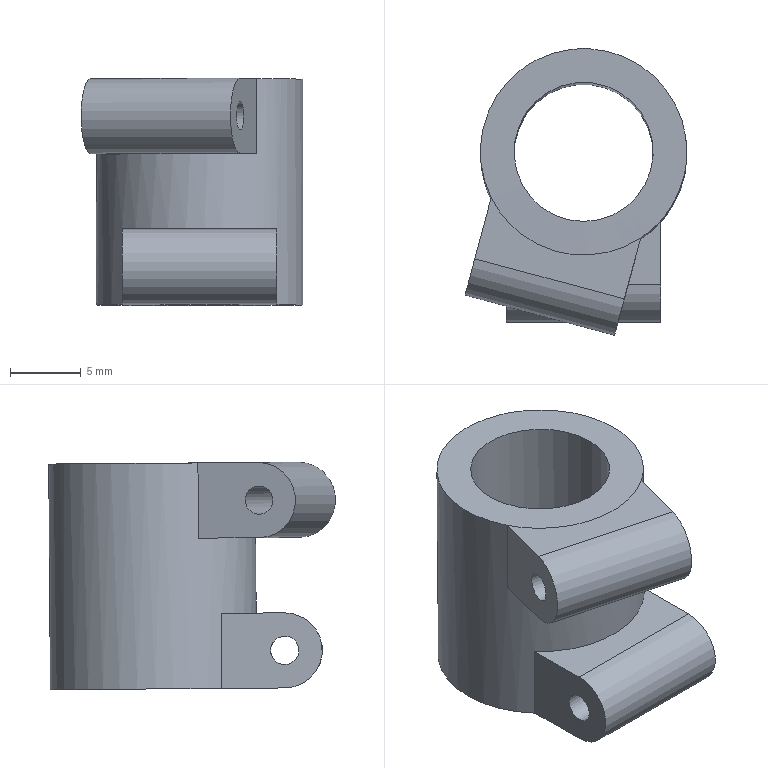Component | NX | CONNECTING_BLOCK | 1 solid | 19 faces | box 15.63 x 20.21 x 16.02 mm | volume 1931 mm3 | plane 13 | cylinder 6 | commonest cylinder face diameters 5.292 x2 2 x2 14.55 x1 9.8 x1
STEP:
#1=VALUE_REPRESENTATION_ITEM('',COUNT_MEASURE(0.));
#2=(LENGTH_UNIT()NAMED_UNIT(*)SI_UNIT(.MILLI.,.METRE.));
#3=UNCERTAINTY_MEASURE_WITH_UNIT(LENGTH_MEASURE(0.0508),#2,'','');
#4=(NAMED_UNIT(*)PLANE_ANGLE_UNIT()SI_UNIT($,.RADIAN.));
#5=PLANE_ANGLE_MEASURE_WITH_UNIT(PLANE_ANGLE_MEASURE(0.01745),#4);
#6=DIMENSIONAL_EXPONENTS(0.,0.,0.,0.,0.,0.,0.);
#7=(CONVERSION_BASED_UNIT('',#5)NAMED_UNIT(#6)PLANE_ANGLE_UNIT());
#8=(NAMED_UNIT(*)SI_UNIT($,.STERADIAN.)SOLID_ANGLE_UNIT());
#9=(GEOMETRIC_REPRESENTATION_CONTEXT(3)GLOBAL_UNCERTAINTY_ASSIGNED_CONTEXT((#3))GLOBAL_UNIT_ASSIGNED_CONTEXT((#2,#7,#8))REPRESENTATION_CONTEXT('',''));
#10=REPRESENTATION('',(#1),#9);
#11=VALUE_REPRESENTATION_ITEM('',COUNT_MEASURE(0.));
#12=REPRESENTATION('',(#11),#9);
#13=CARTESIAN_POINT('',(0.,0.,0.));
#14=DIRECTION('',(0.,0.,1.));
#15=DIRECTION('',(1.,0.,0.));
#16=AXIS2_PLACEMENT_3D('',#13,#14,#15);
#17=SHAPE_REPRESENTATION('',(#16),#9);
#18=CARTESIAN_POINT('',(41.769,-50.521,74.938));
#19=VERTEX_POINT('',#18);
#20=CARTESIAN_POINT('',(52.666,-50.53,74.938));
#21=VERTEX_POINT('',#20);
#22=CARTESIAN_POINT('',(47.221,-45.705,74.902));
#23=DIRECTION('',(0.0000015,0.007573,1.));
#24=DIRECTION('',(0.0007539,1.,-0.007573));
#25=AXIS2_PLACEMENT_3D('',#22,#23,#24);
#26=CIRCLE('',#25,7.275);
#27=EDGE_CURVE('',#19,#21,#26,.T.);
#28=ORIENTED_EDGE('',*,*,#27,.T.);
#29=CARTESIAN_POINT('',(52.666,-50.57,69.647));
#30=VERTEX_POINT('',#29);
#31=CARTESIAN_POINT('',(52.666,-50.57,69.647));
#32=DIRECTION('',(-0.0000015,-0.007573,-1.));
#33=VECTOR('',#32,1.);
#34=LINE('',#31,#33);
#35=EDGE_CURVE('',#21,#30,#34,.T.);
#36=ORIENTED_EDGE('',*,*,#35,.T.);
#37=CARTESIAN_POINT('',(41.769,-50.561,69.647));
#38=VERTEX_POINT('',#37);
#39=CARTESIAN_POINT('',(47.221,-45.745,69.61));
#40=DIRECTION('',(0.0000015,0.007573,1.));
#41=DIRECTION('',(-0.0007539,-1.,0.007573));
#42=AXIS2_PLACEMENT_3D('',#39,#40,#41);
#43=CIRCLE('',#42,7.275);
#44=EDGE_CURVE('',#30,#38,#43,.T.);
#45=ORIENTED_EDGE('',*,*,#44,.T.);
#46=CARTESIAN_POINT('',(41.769,-50.561,69.647));
#47=DIRECTION('',(0.0000015,0.007573,1.));
#48=VECTOR('',#47,1.);
#49=LINE('',#46,#48);
#50=EDGE_CURVE('',#38,#19,#49,.T.);
#51=ORIENTED_EDGE('',*,*,#50,.T.);
#52=EDGE_LOOP('',(#28,#36,#45,#51));
#53=FACE_BOUND('',#52,.T.);
#54=CARTESIAN_POINT('',(40.707,-48.865,85.531));
#55=VERTEX_POINT('',#54);
#56=CARTESIAN_POINT('',(51.233,-51.694,85.553));
#57=VERTEX_POINT('',#56);
#58=CARTESIAN_POINT('',(40.708,-48.865,85.535));
#59=CARTESIAN_POINT('',(40.088,-47.619,85.525));
#60=CARTESIAN_POINT('',(39.836,-46.193,85.514));
#61=CARTESIAN_POINT('',(40.148,-43.428,85.493));
#62=CARTESIAN_POINT('',(40.71,-42.094,85.483));
#63=CARTESIAN_POINT('',(42.472,-39.941,85.467));
#64=CARTESIAN_POINT('',(43.669,-39.125,85.461));
#65=CARTESIAN_POINT('',(46.318,-38.273,85.454));
#66=CARTESIAN_POINT('',(47.766,-38.238,85.454));
#67=CARTESIAN_POINT('',(50.453,-38.96,85.459));
#68=CARTESIAN_POINT('',(51.688,-39.716,85.465));
#69=CARTESIAN_POINT('',(53.553,-41.782,85.481));
#70=CARTESIAN_POINT('',(54.18,-43.087,85.491));
#71=CARTESIAN_POINT('',(54.625,-45.834,85.512));
#72=CARTESIAN_POINT('',(54.443,-47.27,85.522));
#73=CARTESIAN_POINT('',(53.326,-49.819,85.542));
#74=CARTESIAN_POINT('',(52.393,-50.926,85.55));
#75=CARTESIAN_POINT('',(51.233,-51.694,85.556));
#76=B_SPLINE_CURVE_WITH_KNOTS('',3,(#58,#59,#60,#61,#62,#63,#64,#65,#66,#67,#68,#69,#70,#71,#72,#73,#74,#75),.UNSPECIFIED.,.F.,.F.,(4,2,2,2,2,2,2,2,4),(0.,0.125,0.25,0.375,0.5,0.625,0.75,0.875,1.),.UNSPECIFIED.);
#77=EDGE_CURVE('',#55,#57,#76,.T.);
#78=ORIENTED_EDGE('',*,*,#77,.T.);
#79=CARTESIAN_POINT('',(51.232,-51.734,80.256));
#80=VERTEX_POINT('',#79);
#81=CARTESIAN_POINT('',(51.232,-51.815,69.656));
#82=DIRECTION('',(-0.0000015,-0.007573,-1.));
#83=VECTOR('',#82,1.);
#84=LINE('',#81,#83);
#85=EDGE_CURVE('',#57,#80,#84,.T.);
#86=ORIENTED_EDGE('',*,*,#85,.T.);
#87=CARTESIAN_POINT('',(40.708,-48.906,80.235));
#88=VERTEX_POINT('',#87);
#89=CARTESIAN_POINT('',(47.221,-45.665,80.21));
#90=DIRECTION('',(-0.0000015,-0.007573,-1.));
#91=DIRECTION('',(-0.0007539,-1.,0.007573));
#92=AXIS2_PLACEMENT_3D('',#89,#90,#91);
#93=CIRCLE('',#92,7.275);
#94=EDGE_CURVE('',#80,#88,#93,.T.);
#95=ORIENTED_EDGE('',*,*,#94,.T.);
#96=CARTESIAN_POINT('',(40.708,-48.986,69.635));
#97=DIRECTION('',(0.0000015,0.007573,1.));
#98=VECTOR('',#97,1.);
#99=LINE('',#96,#98);
#100=EDGE_CURVE('',#88,#55,#99,.T.);
#101=ORIENTED_EDGE('',*,*,#100,.T.);
#102=EDGE_LOOP('',(#78,#86,#95,#101));
#103=FACE_BOUND('',#102,.T.);
#104=CARTESIAN_POINT('',(47.221,-45.745,69.61));
#105=DIRECTION('',(0.0000015,0.007573,1.));
#106=DIRECTION('',(-0.0007539,-1.,0.007573));
#107=AXIS2_PLACEMENT_3D('',#104,#105,#106);
#108=CYLINDRICAL_SURFACE('',#107,7.275);
#109=ADVANCED_FACE('',(#53,#103),#108,.T.);
#110=CARTESIAN_POINT('',(47.217,-50.525,85.547));
#111=VERTEX_POINT('',#110);
#112=CARTESIAN_POINT('',(47.221,-45.625,85.51));
#113=DIRECTION('',(0.0000015,0.007573,1.));
#114=DIRECTION('',(-0.0007539,-1.,0.007573));
#115=AXIS2_PLACEMENT_3D('',#112,#113,#114);
#116=CIRCLE('',#115,4.9);
#117=EDGE_CURVE('',#111,#111,#116,.T.);
#118=ORIENTED_EDGE('',*,*,#117,.F.);
#119=EDGE_LOOP('',(#118));
#120=FACE_BOUND('',#119,.T.);
#121=CARTESIAN_POINT('',(51.234,-51.693,85.548));
#122=CARTESIAN_POINT('',(49.515,-52.829,85.556));
#123=CARTESIAN_POINT('',(47.323,-53.185,85.559));
#124=CARTESIAN_POINT('',(43.345,-52.116,85.551));
#125=CARTESIAN_POINT('',(41.626,-50.711,85.54));
#126=CARTESIAN_POINT('',(40.708,-48.865,85.526));
#127=B_SPLINE_CURVE_WITH_KNOTS('',3,(#121,#122,#123,#124,#125,#126),.UNSPECIFIED.,.F.,.F.,(4,2,4),(0.,0.5,1.),.UNSPECIFIED.);
#128=EDGE_CURVE('',#57,#55,#127,.T.);
#129=ORIENTED_EDGE('',*,*,#128,.F.);
#130=ORIENTED_EDGE('',*,*,#77,.F.);
#131=EDGE_LOOP('',(#129,#130));
#132=FACE_BOUND('',#131,.T.);
#133=CARTESIAN_POINT('',(47.221,-45.625,85.51));
#134=DIRECTION('',(0.0000015,0.007573,1.));
#135=DIRECTION('',(-0.0007539,-1.,0.007573));
#136=AXIS2_PLACEMENT_3D('',#133,#134,#135);
#137=PLANE('',#136);
#138=ADVANCED_FACE('',(#120,#132),#137,.T.);
#139=CARTESIAN_POINT('',(47.217,-50.645,69.648));
#140=VERTEX_POINT('',#139);
#141=CARTESIAN_POINT('',(47.221,-45.745,69.61));
#142=DIRECTION('',(0.0000015,0.007573,1.));
#143=DIRECTION('',(-0.0007539,-1.,0.007573));
#144=AXIS2_PLACEMENT_3D('',#141,#142,#143);
#145=CIRCLE('',#144,4.9);
#146=EDGE_CURVE('',#140,#140,#145,.T.);
#147=ORIENTED_EDGE('',*,*,#146,.T.);
#148=EDGE_LOOP('',(#147));
#149=FACE_BOUND('',#148,.T.);
#150=ORIENTED_EDGE('',*,*,#44,.F.);
#151=CARTESIAN_POINT('',(52.668,-50.57,69.647));
#152=VERTEX_POINT('',#151);
#153=CARTESIAN_POINT('',(41.768,-50.561,69.647));
#154=DIRECTION('',(1.,-0.0007539,0.00000421));
#155=VECTOR('',#154,1.);
#156=LINE('',#153,#155);
#157=EDGE_CURVE('',#30,#152,#156,.T.);
#158=ORIENTED_EDGE('',*,*,#157,.T.);
#159=CARTESIAN_POINT('',(52.664,-55.009,69.681));
#160=VERTEX_POINT('',#159);
#161=CARTESIAN_POINT('',(52.668,-50.57,69.647));
#162=DIRECTION('',(-0.0007539,-1.,0.007573));
#163=VECTOR('',#162,1.);
#164=LINE('',#161,#163);
#165=EDGE_CURVE('',#152,#160,#164,.T.);
#166=ORIENTED_EDGE('',*,*,#165,.T.);
#167=CARTESIAN_POINT('',(41.764,-55.001,69.681));
#168=VERTEX_POINT('',#167);
#169=CARTESIAN_POINT('',(41.764,-55.001,69.681));
#170=DIRECTION('',(1.,-0.0007539,0.00000421));
#171=VECTOR('',#170,1.);
#172=LINE('',#169,#171);
#173=EDGE_CURVE('',#168,#160,#172,.T.);
#174=ORIENTED_EDGE('',*,*,#173,.F.);
#175=CARTESIAN_POINT('',(41.768,-50.561,69.647));
#176=VERTEX_POINT('',#175);
#177=CARTESIAN_POINT('',(41.768,-50.561,69.647));
#178=DIRECTION('',(-0.0007539,-1.,0.007573));
#179=VECTOR('',#178,1.);
#180=LINE('',#177,#179);
#181=EDGE_CURVE('',#176,#168,#180,.T.);
#182=ORIENTED_EDGE('',*,*,#181,.F.);
#183=CARTESIAN_POINT('',(41.768,-50.561,69.647));
#184=DIRECTION('',(1.,-0.0007539,0.00000421));
#185=VECTOR('',#184,1.);
#186=LINE('',#183,#185);
#187=EDGE_CURVE('',#176,#38,#186,.T.);
#188=ORIENTED_EDGE('',*,*,#187,.T.);
#189=EDGE_LOOP('',(#150,#158,#166,#174,#182,#188));
#190=FACE_BOUND('',#189,.T.);
#191=CARTESIAN_POINT('',(47.221,-45.745,69.61));
#192=DIRECTION('',(-0.0000015,-0.007573,-1.));
#193=DIRECTION('',(0.0007539,1.,-0.007573));
#194=AXIS2_PLACEMENT_3D('',#191,#192,#193);
#195=PLANE('',#194);
#196=ADVANCED_FACE('',(#149,#190),#195,.T.);
#197=ORIENTED_EDGE('',*,*,#35,.F.);
#198=CARTESIAN_POINT('',(52.668,-50.53,74.938));
#199=VERTEX_POINT('',#198);
#200=CARTESIAN_POINT('',(41.768,-50.521,74.938));
#201=DIRECTION('',(1.,-0.0007539,0.00000421));
#202=VECTOR('',#201,1.);
#203=LINE('',#200,#202);
#204=EDGE_CURVE('',#21,#199,#203,.T.);
#205=ORIENTED_EDGE('',*,*,#204,.T.);
#206=CARTESIAN_POINT('',(52.668,-50.53,74.938));
#207=DIRECTION('',(-0.0000015,-0.007573,-1.));
#208=VECTOR('',#207,1.);
#209=LINE('',#206,#208);
#210=EDGE_CURVE('',#199,#152,#209,.T.);
#211=ORIENTED_EDGE('',*,*,#210,.T.);
#212=ORIENTED_EDGE('',*,*,#157,.F.);
#213=EDGE_LOOP('',(#197,#205,#211,#212));
#214=FACE_OUTER_BOUND('',#213,.T.);
#215=CARTESIAN_POINT('',(41.768,-50.521,74.938));
#216=DIRECTION('',(-0.0007539,-1.,0.007573));
#217=DIRECTION('',(-0.0000015,-0.007573,-1.));
#218=AXIS2_PLACEMENT_3D('',#215,#216,#217);
#219=PLANE('',#218);
#220=ADVANCED_FACE('',(#214),#219,.F.);
#221=ORIENTED_EDGE('',*,*,#50,.F.);
#222=ORIENTED_EDGE('',*,*,#187,.F.);
#223=CARTESIAN_POINT('',(41.768,-50.521,74.938));
#224=VERTEX_POINT('',#223);
#225=CARTESIAN_POINT('',(41.768,-50.521,74.938));
#226=DIRECTION('',(-0.0000015,-0.007573,-1.));
#227=VECTOR('',#226,1.);
#228=LINE('',#225,#227);
#229=EDGE_CURVE('',#224,#176,#228,.T.);
#230=ORIENTED_EDGE('',*,*,#229,.F.);
#231=CARTESIAN_POINT('',(41.768,-50.521,74.938));
#232=DIRECTION('',(1.,-0.0007539,0.00000421));
#233=VECTOR('',#232,1.);
#234=LINE('',#231,#233);
#235=EDGE_CURVE('',#224,#19,#234,.T.);
#236=ORIENTED_EDGE('',*,*,#235,.T.);
#237=EDGE_LOOP('',(#221,#222,#230,#236));
#238=FACE_OUTER_BOUND('',#237,.T.);
#239=CARTESIAN_POINT('',(41.768,-50.521,74.938));
#240=DIRECTION('',(-0.0007539,-1.,0.007573));
#241=DIRECTION('',(-0.0000015,-0.007573,-1.));
#242=AXIS2_PLACEMENT_3D('',#239,#240,#241);
#243=PLANE('',#242);
#244=ADVANCED_FACE('',(#238),#243,.F.);
#245=CARTESIAN_POINT('',(52.664,-54.969,74.972));
#246=VERTEX_POINT('',#245);
#247=CARTESIAN_POINT('',(52.664,-54.989,72.326));
#248=DIRECTION('',(-1.,0.0007539,-0.00000421));
#249=DIRECTION('',(0.0000015,0.007573,1.));
#250=AXIS2_PLACEMENT_3D('',#247,#248,#249);
#251=CIRCLE('',#250,2.646);
#252=EDGE_CURVE('',#160,#246,#251,.T.);
#253=ORIENTED_EDGE('',*,*,#252,.T.);
#254=CARTESIAN_POINT('',(41.764,-54.961,74.972));
#255=VERTEX_POINT('',#254);
#256=CARTESIAN_POINT('',(41.764,-54.961,74.972));
#257=DIRECTION('',(1.,-0.0007539,0.00000421));
#258=VECTOR('',#257,1.);
#259=LINE('',#256,#258);
#260=EDGE_CURVE('',#255,#246,#259,.T.);
#261=ORIENTED_EDGE('',*,*,#260,.F.);
#262=CARTESIAN_POINT('',(41.764,-54.981,72.326));
#263=DIRECTION('',(-1.,0.0007539,-0.00000421));
#264=DIRECTION('',(0.0000015,0.007573,1.));
#265=AXIS2_PLACEMENT_3D('',#262,#263,#264);
#266=CIRCLE('',#265,2.646);
#267=EDGE_CURVE('',#168,#255,#266,.T.);
#268=ORIENTED_EDGE('',*,*,#267,.F.);
#269=ORIENTED_EDGE('',*,*,#173,.T.);
#270=EDGE_LOOP('',(#253,#261,#268,#269));
#271=FACE_OUTER_BOUND('',#270,.T.);
#272=CARTESIAN_POINT('',(41.764,-54.981,72.326));
#273=DIRECTION('',(1.,-0.0007539,0.00000421));
#274=DIRECTION('',(0.0000015,0.007573,1.));
#275=AXIS2_PLACEMENT_3D('',#272,#273,#274);
#276=CYLINDRICAL_SURFACE('',#275,2.646);
#277=ADVANCED_FACE('',(#271),#276,.T.);
#278=ORIENTED_EDGE('',*,*,#27,.F.);
#279=ORIENTED_EDGE('',*,*,#235,.F.);
#280=CARTESIAN_POINT('',(41.764,-54.961,74.972));
#281=DIRECTION('',(0.0007539,1.,-0.007573));
#282=VECTOR('',#281,1.);
#283=LINE('',#280,#282);
#284=EDGE_CURVE('',#255,#224,#283,.T.);
#285=ORIENTED_EDGE('',*,*,#284,.F.);
#286=ORIENTED_EDGE('',*,*,#260,.T.);
#287=CARTESIAN_POINT('',(52.664,-54.969,74.972));
#288=DIRECTION('',(0.0007539,1.,-0.007573));
#289=VECTOR('',#288,1.);
#290=LINE('',#287,#289);
#291=EDGE_CURVE('',#246,#199,#290,.T.);
#292=ORIENTED_EDGE('',*,*,#291,.T.);
#293=ORIENTED_EDGE('',*,*,#204,.F.);
#294=EDGE_LOOP('',(#278,#279,#285,#286,#292,#293));
#295=FACE_OUTER_BOUND('',#294,.T.);
#296=CARTESIAN_POINT('',(41.764,-54.961,74.972));
#297=DIRECTION('',(-0.0000015,-0.007573,-1.));
#298=DIRECTION('',(0.0007539,1.,-0.007573));
#299=AXIS2_PLACEMENT_3D('',#296,#297,#298);
#300=PLANE('',#299);
#301=ADVANCED_FACE('',(#295),#300,.F.);
#302=CARTESIAN_POINT('',(41.764,-54.974,73.326));
#303=VERTEX_POINT('',#302);
#304=CARTESIAN_POINT('',(41.764,-54.981,72.326));
#305=DIRECTION('',(1.,-0.0007539,0.00000421));
#306=DIRECTION('',(0.0000015,0.007573,1.));
#307=AXIS2_PLACEMENT_3D('',#304,#305,#306);
#308=CIRCLE('',#307,1.);
#309=EDGE_CURVE('',#303,#303,#308,.T.);
#310=ORIENTED_EDGE('',*,*,#309,.T.);
#311=EDGE_LOOP('',(#310));
#312=FACE_BOUND('',#311,.T.);
#313=ORIENTED_EDGE('',*,*,#229,.T.);
#314=ORIENTED_EDGE('',*,*,#181,.T.);
#315=ORIENTED_EDGE('',*,*,#267,.T.);
#316=ORIENTED_EDGE('',*,*,#284,.T.);
#317=EDGE_LOOP('',(#313,#314,#315,#316));
#318=FACE_BOUND('',#317,.T.);
#319=CARTESIAN_POINT('',(41.764,-54.981,72.326));
#320=DIRECTION('',(-1.,0.0007539,-0.00000421));
#321=DIRECTION('',(-0.0000015,-0.007573,-1.));
#322=AXIS2_PLACEMENT_3D('',#319,#320,#321);
#323=PLANE('',#322);
#324=ADVANCED_FACE('',(#312,#318),#323,.T.);
#325=CARTESIAN_POINT('',(52.664,-54.997,71.326));
#326=VERTEX_POINT('',#325);
#327=CARTESIAN_POINT('',(52.664,-54.989,72.326));
#328=DIRECTION('',(-1.,0.0007539,-0.00000421));
#329=DIRECTION('',(-0.0000015,-0.007573,-1.));
#330=AXIS2_PLACEMENT_3D('',#327,#328,#329);
#331=CIRCLE('',#330,1.);
#332=EDGE_CURVE('',#326,#326,#331,.T.);
#333=ORIENTED_EDGE('',*,*,#332,.T.);
#334=EDGE_LOOP('',(#333));
#335=FACE_BOUND('',#334,.T.);
#336=ORIENTED_EDGE('',*,*,#210,.F.);
#337=ORIENTED_EDGE('',*,*,#291,.F.);
#338=ORIENTED_EDGE('',*,*,#252,.F.);
#339=ORIENTED_EDGE('',*,*,#165,.F.);
#340=EDGE_LOOP('',(#336,#337,#338,#339));
#341=FACE_BOUND('',#340,.T.);
#342=CARTESIAN_POINT('',(52.664,-54.989,72.326));
#343=DIRECTION('',(-1.,0.0007539,-0.00000421));
#344=DIRECTION('',(-0.0000015,-0.007573,-1.));
#345=AXIS2_PLACEMENT_3D('',#342,#343,#344);
#346=PLANE('',#345);
#347=ADVANCED_FACE('',(#335,#341),#346,.F.);
#348=CARTESIAN_POINT('',(50.081,-55.982,85.58));
#349=VERTEX_POINT('',#348);
#350=CARTESIAN_POINT('',(50.081,-55.982,85.58));
#351=DIRECTION('',(0.2595,0.9657,-0.007314));
#352=VECTOR('',#351,1.);
#353=LINE('',#350,#352);
#354=EDGE_CURVE('',#349,#57,#353,.T.);
#355=ORIENTED_EDGE('',*,*,#354,.T.);
#356=ORIENTED_EDGE('',*,*,#128,.T.);
#357=CARTESIAN_POINT('',(39.554,-53.153,85.559));
#358=VERTEX_POINT('',#357);
#359=CARTESIAN_POINT('',(39.554,-53.153,85.559));
#360=DIRECTION('',(0.2595,0.9657,-0.007314));
#361=VECTOR('',#360,1.);
#362=LINE('',#359,#361);
#363=EDGE_CURVE('',#358,#55,#362,.T.);
#364=ORIENTED_EDGE('',*,*,#363,.F.);
#365=CARTESIAN_POINT('',(39.554,-53.153,85.559));
#366=DIRECTION('',(0.9657,-0.2595,0.001964));
#367=VECTOR('',#366,1.);
#368=LINE('',#365,#367);
#369=EDGE_CURVE('',#358,#349,#368,.T.);
#370=ORIENTED_EDGE('',*,*,#369,.T.);
#371=EDGE_LOOP('',(#355,#356,#364,#370));
#372=FACE_OUTER_BOUND('',#371,.T.);
#373=CARTESIAN_POINT('',(39.554,-53.153,85.559));
#374=DIRECTION('',(-0.0000015,-0.007573,-1.));
#375=DIRECTION('',(0.2595,0.9657,-0.007314));
#376=AXIS2_PLACEMENT_3D('',#373,#374,#375);
#377=PLANE('',#376);
#378=ADVANCED_FACE('',(#372),#377,.F.);
#379=ORIENTED_EDGE('',*,*,#85,.F.);
#380=CARTESIAN_POINT('',(51.233,-51.735,80.256));
#381=VERTEX_POINT('',#380);
#382=CARTESIAN_POINT('',(51.233,-51.695,85.548));
#383=DIRECTION('',(-0.0000015,-0.007573,-1.));
#384=VECTOR('',#383,1.);
#385=LINE('',#382,#384);
#386=EDGE_CURVE('',#57,#381,#385,.T.);
#387=ORIENTED_EDGE('',*,*,#386,.T.);
#388=CARTESIAN_POINT('',(40.707,-48.906,80.235));
#389=DIRECTION('',(0.9657,-0.2595,0.001964));
#390=VECTOR('',#389,1.);
#391=LINE('',#388,#390);
#392=EDGE_CURVE('',#80,#381,#391,.T.);
#393=ORIENTED_EDGE('',*,*,#392,.F.);
#394=EDGE_LOOP('',(#379,#387,#393));
#395=FACE_OUTER_BOUND('',#394,.T.);
#396=CARTESIAN_POINT('',(40.707,-48.866,85.526));
#397=DIRECTION('',(-0.2595,-0.9657,0.007314));
#398=DIRECTION('',(-0.0000015,-0.007573,-1.));
#399=AXIS2_PLACEMENT_3D('',#396,#397,#398);
#400=PLANE('',#399);
#401=ADVANCED_FACE('',(#395),#400,.F.);
#402=ORIENTED_EDGE('',*,*,#100,.F.);
#403=CARTESIAN_POINT('',(40.707,-48.906,80.235));
#404=VERTEX_POINT('',#403);
#405=CARTESIAN_POINT('',(40.707,-48.906,80.235));
#406=DIRECTION('',(0.9657,-0.2595,0.001964));
#407=VECTOR('',#406,1.);
#408=LINE('',#405,#407);
#409=EDGE_CURVE('',#404,#88,#408,.T.);
#410=ORIENTED_EDGE('',*,*,#409,.F.);
#411=CARTESIAN_POINT('',(40.707,-48.866,85.526));
#412=DIRECTION('',(-0.0000015,-0.007573,-1.));
#413=VECTOR('',#412,1.);
#414=LINE('',#411,#413);
#415=EDGE_CURVE('',#55,#404,#414,.T.);
#416=ORIENTED_EDGE('',*,*,#415,.F.);
#417=EDGE_LOOP('',(#402,#410,#416));
#418=FACE_OUTER_BOUND('',#417,.T.);
#419=CARTESIAN_POINT('',(40.707,-48.866,85.526));
#420=DIRECTION('',(-0.2595,-0.9657,0.007314));
#421=DIRECTION('',(-0.0000015,-0.007573,-1.));
#422=AXIS2_PLACEMENT_3D('',#419,#420,#421);
#423=PLANE('',#422);
#424=ADVANCED_FACE('',(#418),#423,.F.);
#425=ORIENTED_EDGE('',*,*,#94,.F.);
#426=ORIENTED_EDGE('',*,*,#392,.T.);
#427=CARTESIAN_POINT('',(50.081,-56.022,80.289));
#428=VERTEX_POINT('',#427);
#429=CARTESIAN_POINT('',(51.233,-51.735,80.256));
#430=DIRECTION('',(-0.2595,-0.9657,0.007314));
#431=VECTOR('',#430,1.);
#432=LINE('',#429,#431);
#433=EDGE_CURVE('',#381,#428,#432,.T.);
#434=ORIENTED_EDGE('',*,*,#433,.T.);
#435=CARTESIAN_POINT('',(39.554,-53.193,80.267));
#436=VERTEX_POINT('',#435);
#437=CARTESIAN_POINT('',(39.554,-53.193,80.267));
#438=DIRECTION('',(0.9657,-0.2595,0.001964));
#439=VECTOR('',#438,1.);
#440=LINE('',#437,#439);
#441=EDGE_CURVE('',#436,#428,#440,.T.);
#442=ORIENTED_EDGE('',*,*,#441,.F.);
#443=CARTESIAN_POINT('',(40.707,-48.906,80.235));
#444=DIRECTION('',(-0.2595,-0.9657,0.007314));
#445=VECTOR('',#444,1.);
#446=LINE('',#443,#445);
#447=EDGE_CURVE('',#404,#436,#446,.T.);
#448=ORIENTED_EDGE('',*,*,#447,.F.);
#449=ORIENTED_EDGE('',*,*,#409,.T.);
#450=EDGE_LOOP('',(#425,#426,#434,#442,#448,#449));
#451=FACE_OUTER_BOUND('',#450,.T.);
#452=CARTESIAN_POINT('',(40.707,-48.906,80.235));
#453=DIRECTION('',(0.0000015,0.007573,1.));
#454=DIRECTION('',(-0.2595,-0.9657,0.007314));
#455=AXIS2_PLACEMENT_3D('',#452,#453,#454);
#456=PLANE('',#455);
#457=ADVANCED_FACE('',(#451),#456,.F.);
#458=CARTESIAN_POINT('',(50.081,-56.002,82.934));
#459=DIRECTION('',(-0.9657,0.2595,-0.001964));
#460=DIRECTION('',(0.0000015,0.007573,1.));
#461=AXIS2_PLACEMENT_3D('',#458,#459,#460);
#462=CIRCLE('',#461,2.646);
#463=EDGE_CURVE('',#428,#349,#462,.T.);
#464=ORIENTED_EDGE('',*,*,#463,.T.);
#465=ORIENTED_EDGE('',*,*,#369,.F.);
#466=CARTESIAN_POINT('',(39.554,-53.173,82.913));
#467=DIRECTION('',(-0.9657,0.2595,-0.001964));
#468=DIRECTION('',(0.0000015,0.007573,1.));
#469=AXIS2_PLACEMENT_3D('',#466,#467,#468);
#470=CIRCLE('',#469,2.646);
#471=EDGE_CURVE('',#436,#358,#470,.T.);
#472=ORIENTED_EDGE('',*,*,#471,.F.);
#473=ORIENTED_EDGE('',*,*,#441,.T.);
#474=EDGE_LOOP('',(#464,#465,#472,#473));
#475=FACE_OUTER_BOUND('',#474,.T.);
#476=CARTESIAN_POINT('',(39.554,-53.173,82.913));
#477=DIRECTION('',(0.9657,-0.2595,0.001964));
#478=DIRECTION('',(0.0000015,0.007573,1.));
#479=AXIS2_PLACEMENT_3D('',#476,#477,#478);
#480=CYLINDRICAL_SURFACE('',#479,2.646);
#481=ADVANCED_FACE('',(#475),#480,.T.);
#482=CARTESIAN_POINT('',(39.814,-52.207,82.906));
#483=VERTEX_POINT('',#482);
#484=CARTESIAN_POINT('',(39.554,-53.173,82.913));
#485=DIRECTION('',(0.9657,-0.2595,0.001964));
#486=DIRECTION('',(0.2595,0.9657,-0.007314));
#487=AXIS2_PLACEMENT_3D('',#484,#485,#486);
#488=CIRCLE('',#487,1.);
#489=EDGE_CURVE('',#483,#483,#488,.T.);
#490=ORIENTED_EDGE('',*,*,#489,.T.);
#491=EDGE_LOOP('',(#490));
#492=FACE_BOUND('',#491,.T.);
#493=ORIENTED_EDGE('',*,*,#415,.T.);
#494=ORIENTED_EDGE('',*,*,#447,.T.);
#495=ORIENTED_EDGE('',*,*,#471,.T.);
#496=ORIENTED_EDGE('',*,*,#363,.T.);
#497=EDGE_LOOP('',(#493,#494,#495,#496));
#498=FACE_BOUND('',#497,.T.);
#499=CARTESIAN_POINT('',(39.554,-53.173,82.913));
#500=DIRECTION('',(-0.9657,0.2595,-0.001964));
#501=DIRECTION('',(-0.0000015,-0.007573,-1.));
#502=AXIS2_PLACEMENT_3D('',#499,#500,#501);
#503=PLANE('',#502);
#504=ADVANCED_FACE('',(#492,#498),#503,.T.);
#505=CARTESIAN_POINT('',(49.821,-56.968,82.942));
#506=VERTEX_POINT('',#505);
#507=CARTESIAN_POINT('',(50.081,-56.002,82.934));
#508=DIRECTION('',(-0.9657,0.2595,-0.001964));
#509=DIRECTION('',(-0.2595,-0.9657,0.007314));
#510=AXIS2_PLACEMENT_3D('',#507,#508,#509);
#511=CIRCLE('',#510,1.);
#512=EDGE_CURVE('',#506,#506,#511,.T.);
#513=ORIENTED_EDGE('',*,*,#512,.T.);
#514=EDGE_LOOP('',(#513));
#515=FACE_BOUND('',#514,.T.);
#516=ORIENTED_EDGE('',*,*,#386,.F.);
#517=ORIENTED_EDGE('',*,*,#354,.F.);
#518=ORIENTED_EDGE('',*,*,#463,.F.);
#519=ORIENTED_EDGE('',*,*,#433,.F.);
#520=EDGE_LOOP('',(#516,#517,#518,#519));
#521=FACE_BOUND('',#520,.T.);
#522=CARTESIAN_POINT('',(50.081,-56.002,82.934));
#523=DIRECTION('',(-0.9657,0.2595,-0.001964));
#524=DIRECTION('',(-0.0000015,-0.007573,-1.));
#525=AXIS2_PLACEMENT_3D('',#522,#523,#524);
#526=PLANE('',#525);
#527=ADVANCED_FACE('',(#515,#521),#526,.F.);
#528=ORIENTED_EDGE('',*,*,#489,.F.);
#529=EDGE_LOOP('',(#528));
#530=FACE_BOUND('',#529,.T.);
#531=ORIENTED_EDGE('',*,*,#512,.F.);
#532=EDGE_LOOP('',(#531));
#533=FACE_BOUND('',#532,.T.);
#534=CARTESIAN_POINT('',(39.554,-53.173,82.913));
#535=DIRECTION('',(0.9657,-0.2595,0.001964));
#536=DIRECTION('',(0.2595,0.9657,-0.007314));
#537=AXIS2_PLACEMENT_3D('',#534,#535,#536);
#538=CYLINDRICAL_SURFACE('',#537,1.);
#539=ADVANCED_FACE('',(#530,#533),#538,.F.);
#540=ORIENTED_EDGE('',*,*,#309,.F.);
#541=EDGE_LOOP('',(#540));
#542=FACE_BOUND('',#541,.T.);
#543=ORIENTED_EDGE('',*,*,#332,.F.);
#544=EDGE_LOOP('',(#543));
#545=FACE_BOUND('',#544,.T.);
#546=CARTESIAN_POINT('',(41.764,-54.981,72.326));
#547=DIRECTION('',(1.,-0.0007539,0.00000421));
#548=DIRECTION('',(0.0000015,0.007573,1.));
#549=AXIS2_PLACEMENT_3D('',#546,#547,#548);
#550=CYLINDRICAL_SURFACE('',#549,1.);
#551=ADVANCED_FACE('',(#542,#545),#550,.F.);
#552=ORIENTED_EDGE('',*,*,#117,.T.);
#553=EDGE_LOOP('',(#552));
#554=FACE_BOUND('',#553,.T.);
#555=ORIENTED_EDGE('',*,*,#146,.F.);
#556=EDGE_LOOP('',(#555));
#557=FACE_BOUND('',#556,.T.);
#558=CARTESIAN_POINT('',(47.221,-45.745,69.61));
#559=DIRECTION('',(0.0000015,0.007573,1.));
#560=DIRECTION('',(-0.0007539,-1.,0.007573));
#561=AXIS2_PLACEMENT_3D('',#558,#559,#560);
#562=CYLINDRICAL_SURFACE('',#561,4.9);
#563=ADVANCED_FACE('',(#554,#557),#562,.F.);
#564=CLOSED_SHELL('',(#109,#138,#196,#220,#244,#277,#301,#324,#347,#378,#401,#424,#457,#481,#504,#527,#539,#551,#563));
#565=MANIFOLD_SOLID_BREP('',#564);
#566=ADVANCED_BREP_SHAPE_REPRESENTATION('',(#565),#9);
#567=SHAPE_REPRESENTATION_RELATIONSHIP('','',#17,#566);
#568=PRESENTATION_LAYER_ASSIGNMENT('','',(#565));
#569=COLOUR_RGB('',0.5961,0.6667,0.6863);
#570=FILL_AREA_STYLE_COLOUR('',#569);
#571=FILL_AREA_STYLE('',(#570));
#572=SURFACE_STYLE_FILL_AREA(#571);
#573=SURFACE_SIDE_STYLE('',(#572));
#574=SURFACE_STYLE_USAGE(.BOTH.,#573);
#575=PRESENTATION_STYLE_ASSIGNMENT((#574));
#576=STYLED_ITEM('',(#575),#565);
#577=MECHANICAL_DESIGN_GEOMETRIC_PRESENTATION_REPRESENTATION('',(#576),#9);